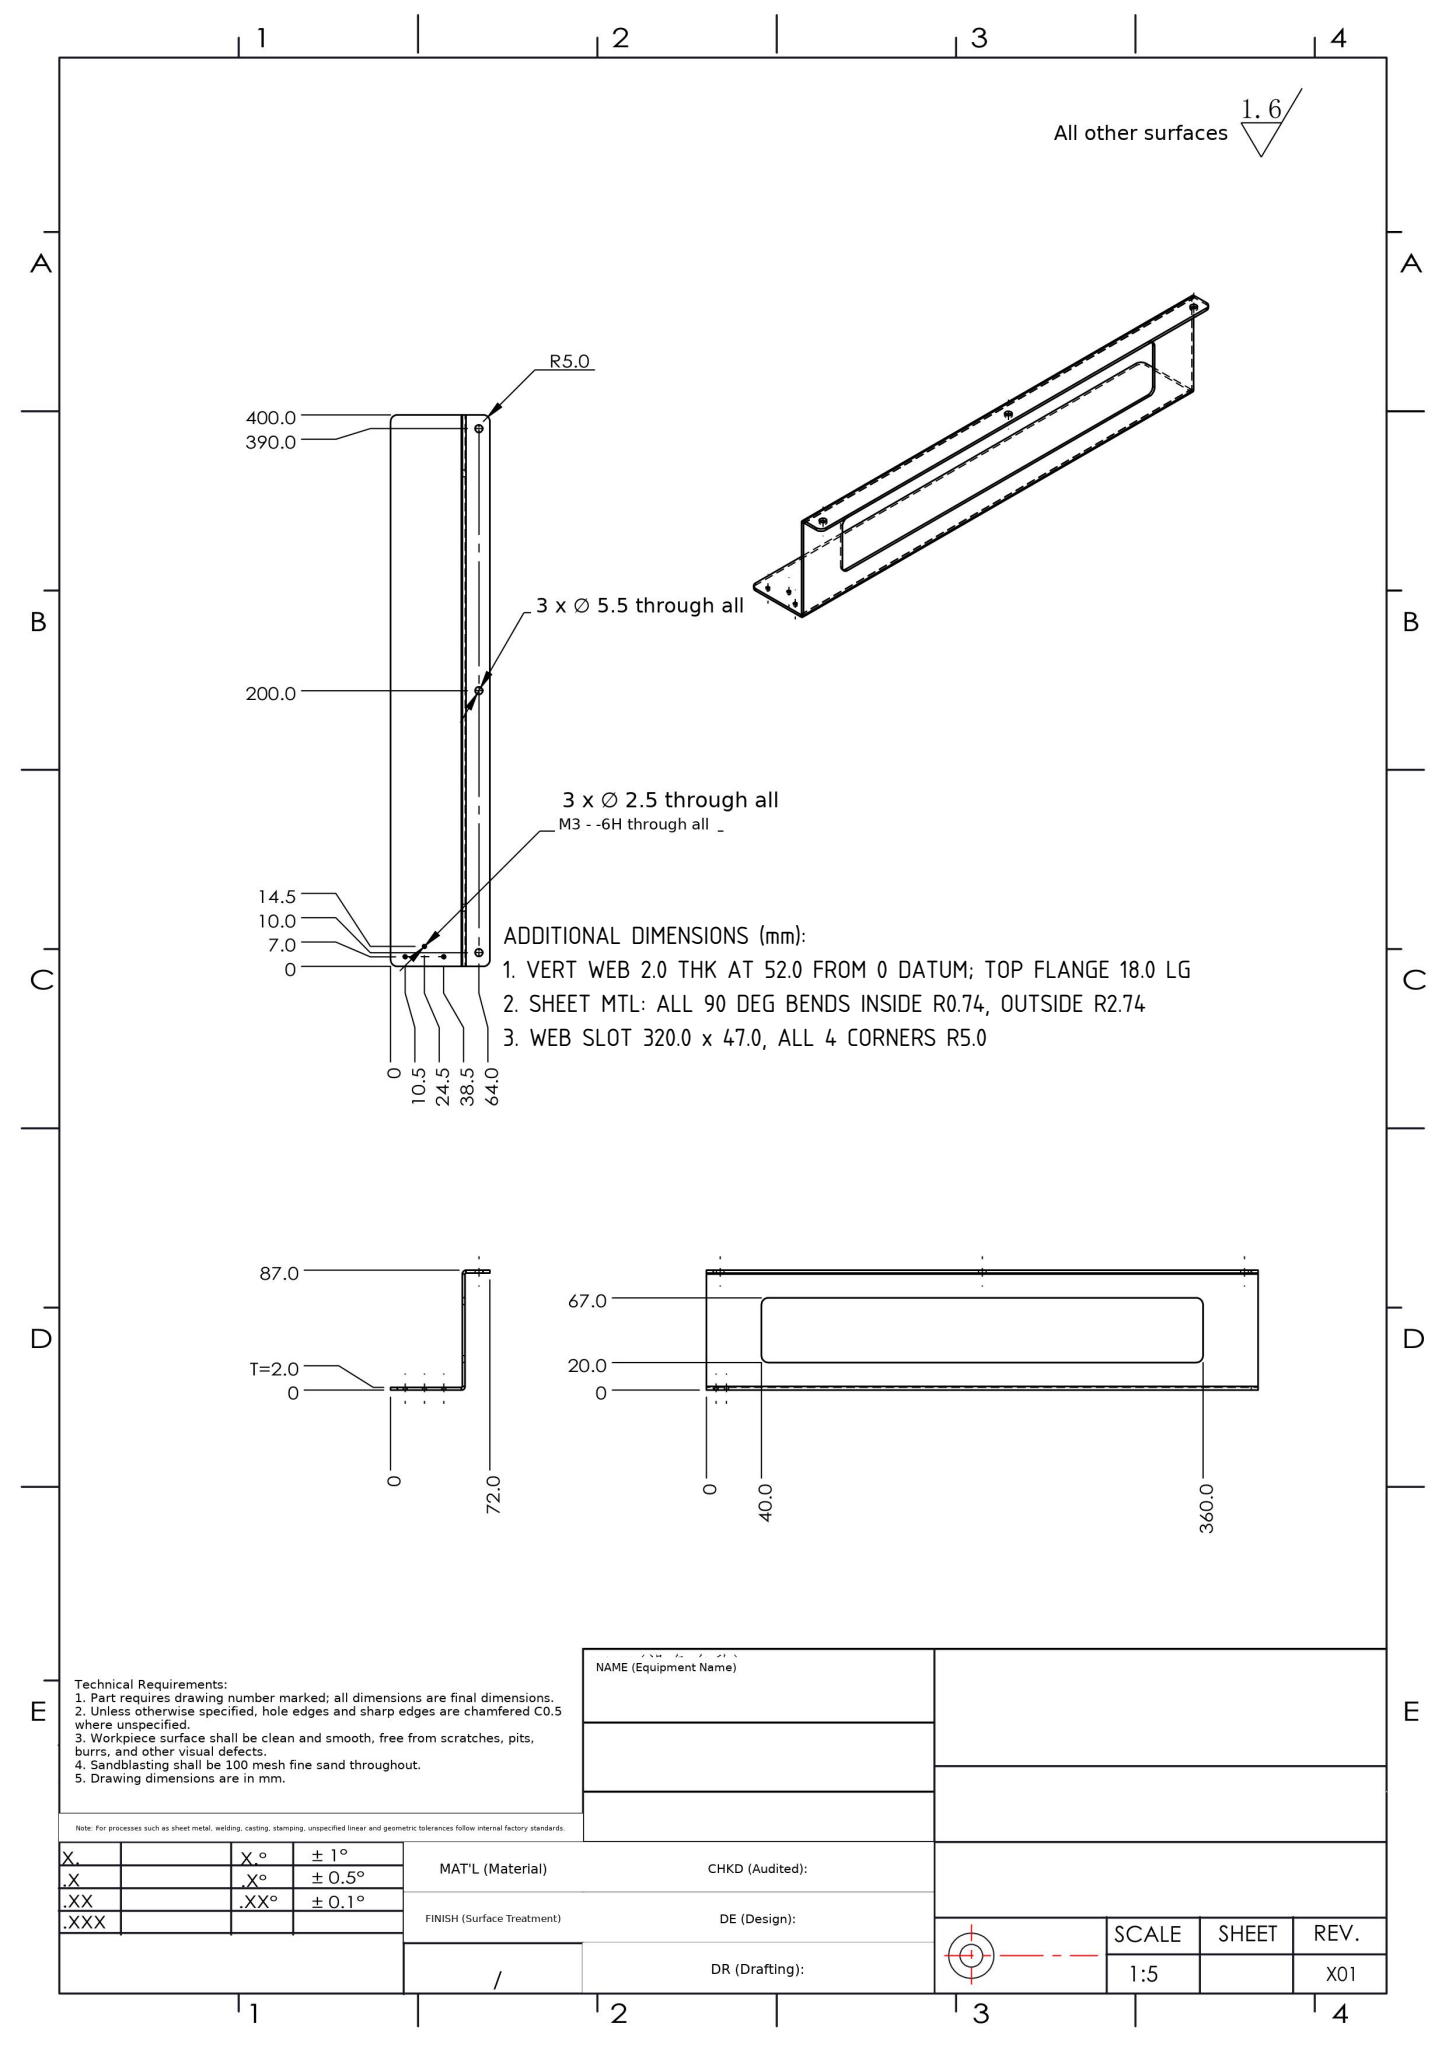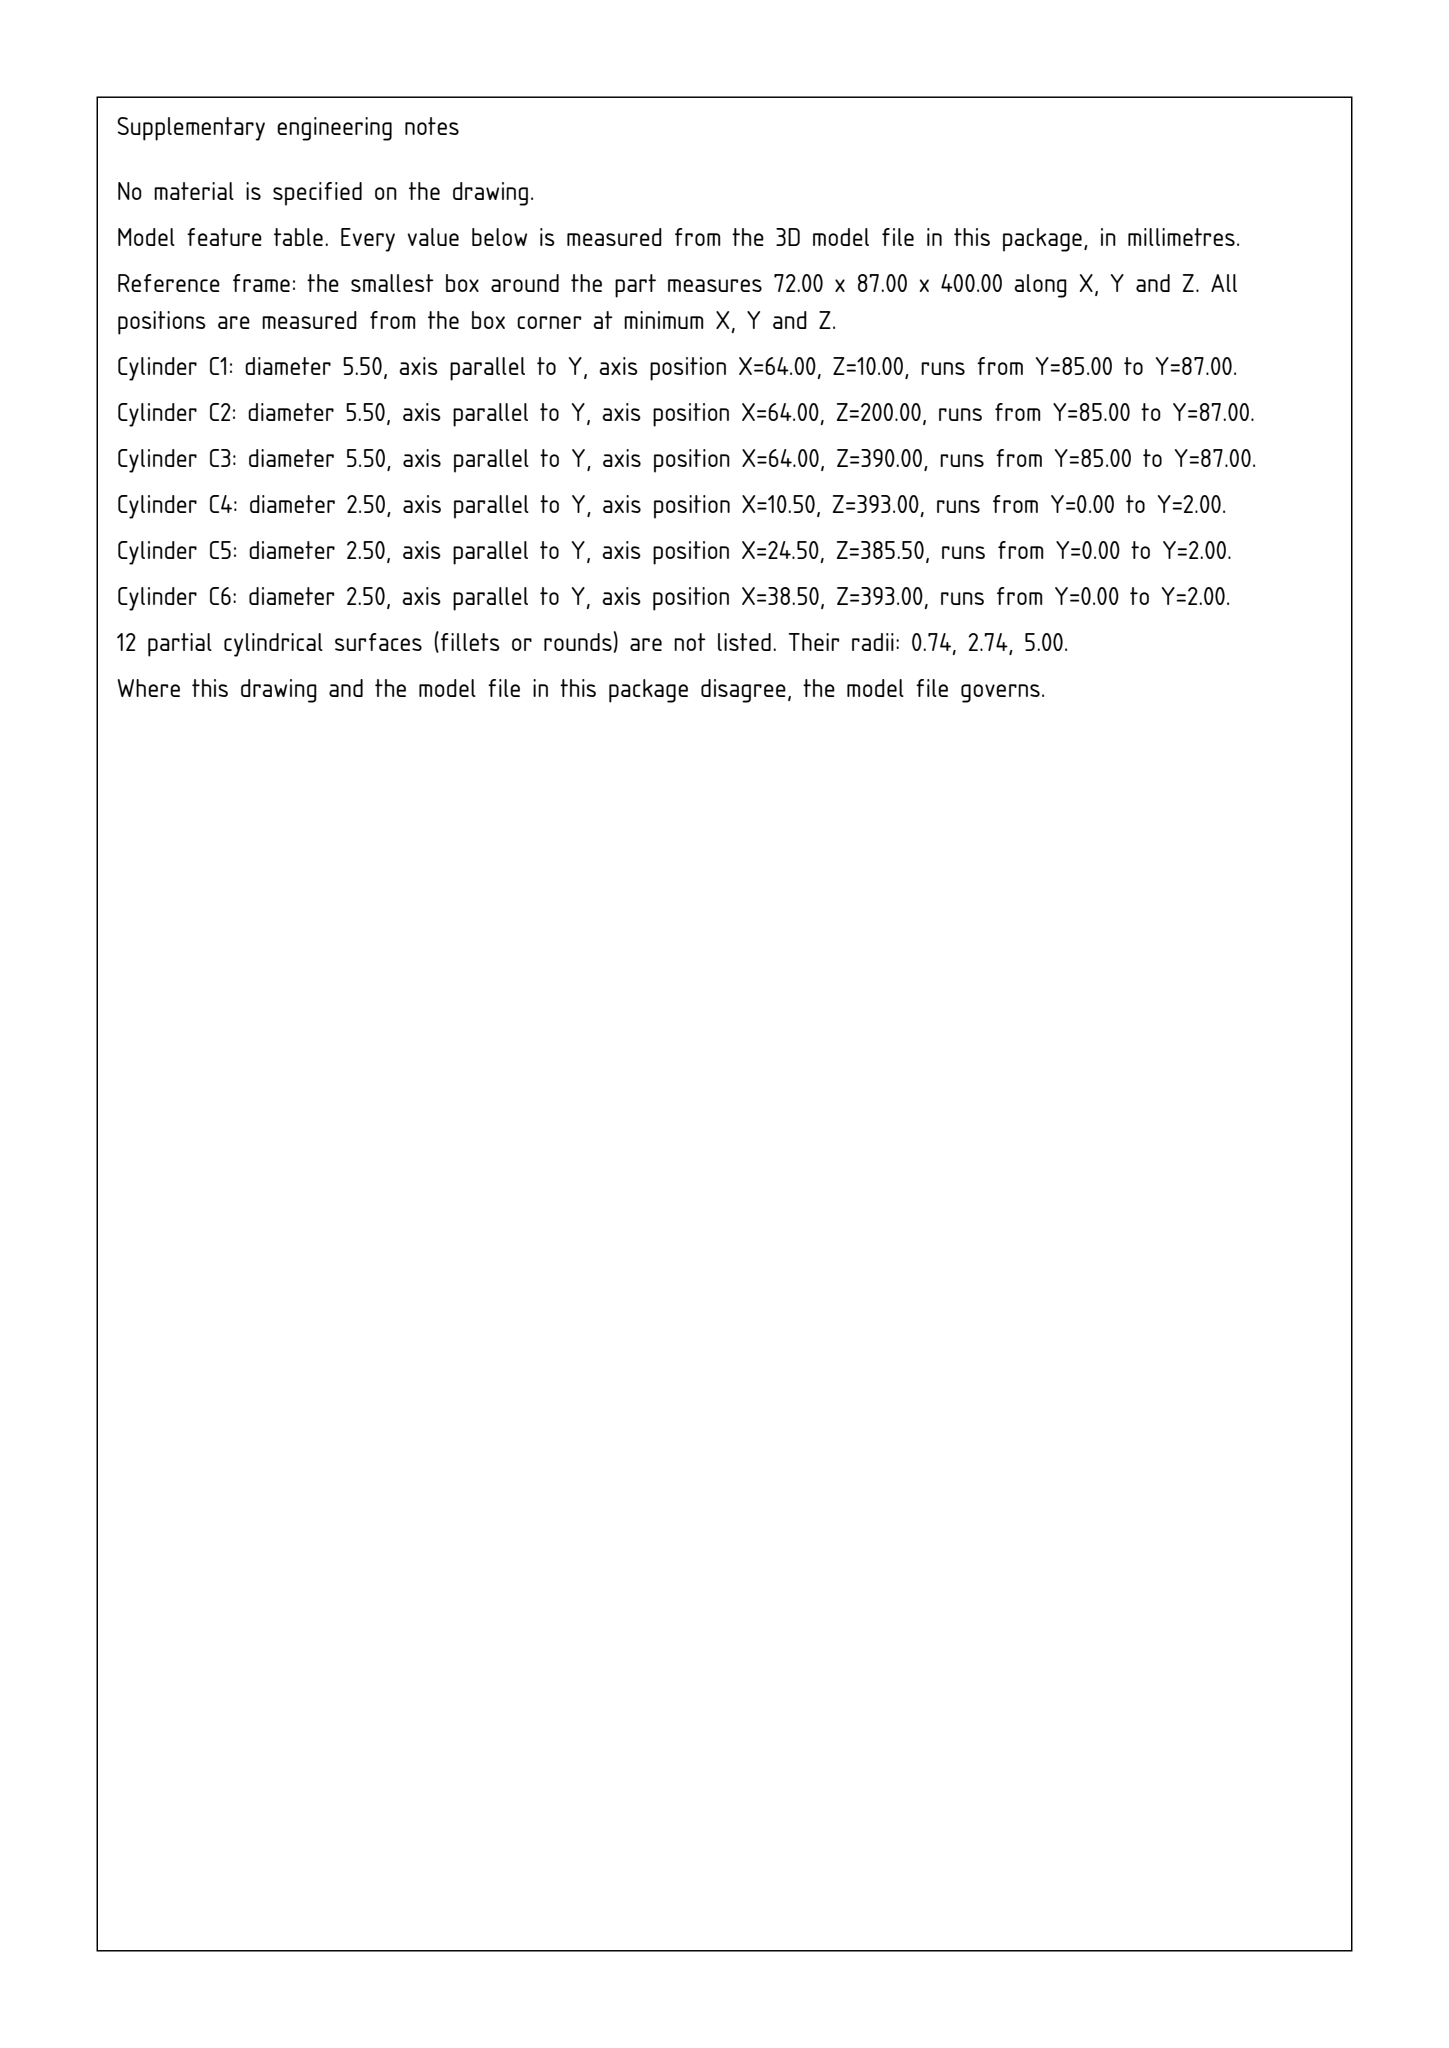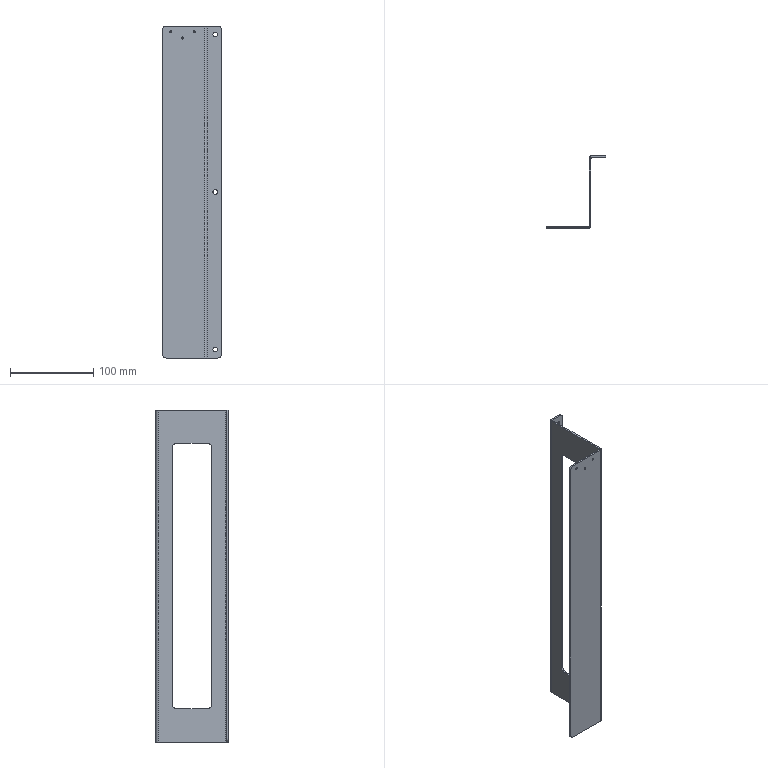Part | SolidWorks | mm | 1 solid | 46 faces | box 72 x 87 x 400 mm | volume 94155 mm3 | cylinder 24 | plane 22 | commonest cylinder face diameters 10 x8 2.5 x6 5.5 x6 5.473 x2 1.473 x2